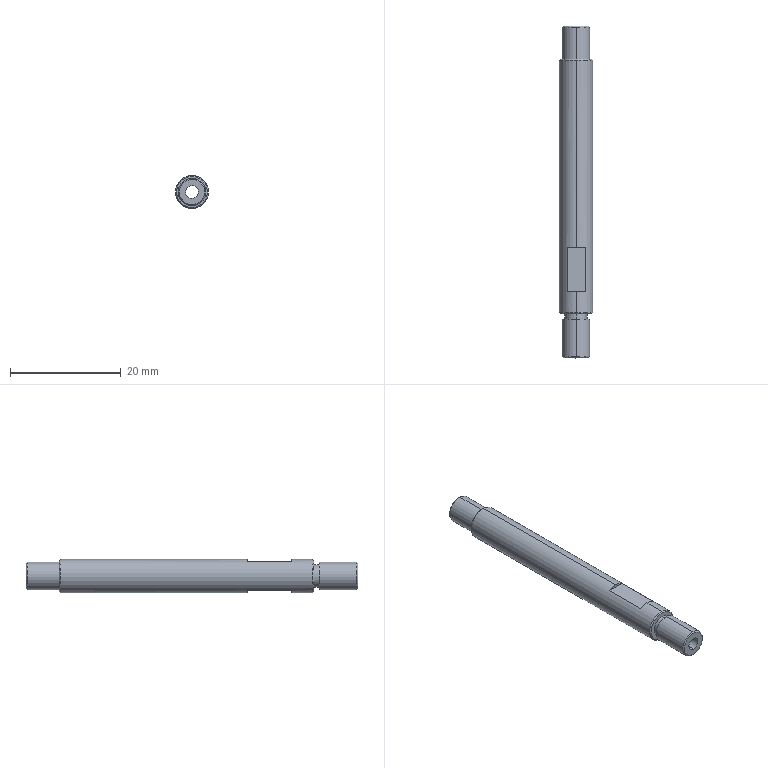Component | SolidWorks | F12529-M5106-1 | 1 solid | 29 faces | box 6 x 60 x 6 mm | volume 1300 mm3 | plane 11 | cylinder 10 | cone 8 | commonest cylinder face diameters 5 x4 2.3 x2 4 x2 6 x2 | material AISI 304
build123d program:
from build123d import *

# Parameters (mm, degrees)
SKETCH2_R          = 3
EXTRUDE1_DEPTH     = 52
SKETCH6_OUTSIDE_W  = 18.538
SKETCH6_OUTSIDE_H  = 18.538
SKETCH6_OUTSIDE_R  = 2.5
CUT_EXTRUDE2_DEPTH = 6
SKETCH7_R          = 2.5
EXTRUDE2_DEPTH     = 8
CHAMFER1_SIZE      = 0.2
SKETCH8_OUTSIDE_W  = 20.12
SKETCH8_OUTSIDE_H  = 20.12
SKETCH8_OUTSIDE_R  = 2
CUT_EXTRUDE3_DEPTH = 1
SKETCH9_R          = 1.15
CUT_EXTRUDE4_DEPTH = 61.15
CUT_EXTRUDE5_START = 2.5
SKETCH10_W         = 8
SKETCH10_H         = 8
CUT_EXTRUDE5_DEPTH = 10


with BuildPart() as part:
    # Sketch2 → Extrude1 (new body)
    with BuildSketch(Plane(origin=(0, 0, 0), x_dir=(1, 0, 0), z_dir=(0, 1, 0))):
        with Locations(Location((0, 0, 0), (0, 0, 90))):
            Circle(SKETCH2_R)
    extrude(amount=EXTRUDE1_DEPTH)

    # Sketch6 outside → Cut-Extrude2 (cut)
    with BuildSketch(Plane(origin=(0, 52, 0), x_dir=(1, 0, 0), z_dir=(0, 1, 0))):
        Rectangle(SKETCH6_OUTSIDE_W, SKETCH6_OUTSIDE_H)
        with Locations(Location((0, 0, 0), (0, 0, 270))):
            Circle(SKETCH6_OUTSIDE_R, mode=Mode.SUBTRACT)
    extrude(amount=-CUT_EXTRUDE2_DEPTH, mode=Mode.SUBTRACT)

    # Sketch7 → Extrude2 (add)
    with BuildSketch(Plane.XZ):
        with Locations(Location((0, 0, 0), (0, 0, 90))):
            Circle(SKETCH7_R)
    extrude(amount=EXTRUDE2_DEPTH)

    # Chamfer1
    chamfer1_edges = [part.edges().sort_by_distance(p)[0] for p in [
        (0, 52, -2.5),
        (0, 0, 3),
        (0, -8, -2.5),
        (0, 46, 3),
    ]]
    chamfer(chamfer1_edges, length=CHAMFER1_SIZE)

    # Sketch8 outside → Cut-Extrude3 (cut)
    with BuildSketch(Plane.XZ):
        Rectangle(SKETCH8_OUTSIDE_W, SKETCH8_OUTSIDE_H)
        with Locations(Location((0, 0, 0), (0, 0, 270))):
            Circle(SKETCH8_OUTSIDE_R, mode=Mode.SUBTRACT)
    extrude(amount=CUT_EXTRUDE3_DEPTH, mode=Mode.SUBTRACT)

    # Sketch9 → Cut-Extrude4 (cut, through all)
    with BuildSketch(Plane(origin=(0, 52, 0), x_dir=(1, 0, 0), z_dir=(0, 1, 0))):
        with Locations(Location((0, 0, 0), (0, 0, 270))):
            Circle(SKETCH9_R)
    extrude(amount=-CUT_EXTRUDE4_DEPTH, mode=Mode.SUBTRACT)

    # Sketch10 → Cut-Extrude5 (cut)
    with BuildSketch(Plane.XY.offset(CUT_EXTRUDE5_START)):
        with Locations((0, 8)):
            Rectangle(SKETCH10_W, SKETCH10_H)
    cut_extrude5 = extrude(amount=CUT_EXTRUDE5_DEPTH, mode=Mode.SUBTRACT)

    # Mirror1: Cut-Extrude5 across plane
    add(cut_extrude5.mirror(Plane.XY), mode=Mode.SUBTRACT)


solid = part.part

# Placed as in the assembly
solid = solid.moved(Location((-17.5, 227.5, 10), (180, -2.312, 180)))
STEP:
#1=CARTESIAN_POINT('',(-0.6908,8.642,0.3485));
#2=VERTEX_POINT('',#1);
#3=CARTESIAN_POINT('',(-0.6871,8.642,0.4389));
#4=VERTEX_POINT('',#3);
#5=CARTESIAN_POINT('',(-0.689,8.642,0.3937));
#6=DIRECTION('',(0.,1.,-0.));
#7=DIRECTION('',(0.04034,0.,0.9992));
#8=AXIS2_PLACEMENT_3D('',#5,#6,#7);
#9=CIRCLE('',#8,0.04528);
#10=EDGE_CURVE('',#2,#4,#9,.T.);
#11=ORIENTED_EDGE('',*,*,#10,.F.);
#12=CARTESIAN_POINT('',(-0.6908,11.004,0.3485));
#13=VERTEX_POINT('',#12);
#14=CARTESIAN_POINT('',(-0.6908,8.642,0.3485));
#15=DIRECTION('',(0.,1.,-0.));
#16=VECTOR('',#15,39.37);
#17=LINE('',#14,#16);
#18=EDGE_CURVE('',#2,#13,#17,.T.);
#19=ORIENTED_EDGE('',*,*,#18,.T.);
#20=CARTESIAN_POINT('',(-0.6871,11.004,0.4389));
#21=VERTEX_POINT('',#20);
#22=CARTESIAN_POINT('',(-0.689,11.004,0.3937));
#23=DIRECTION('',(0.,1.,-0.));
#24=DIRECTION('',(0.04034,0.,0.9992));
#25=AXIS2_PLACEMENT_3D('',#22,#23,#24);
#26=CIRCLE('',#25,0.04528);
#27=EDGE_CURVE('',#13,#21,#26,.T.);
#28=ORIENTED_EDGE('',*,*,#27,.T.);
#29=CARTESIAN_POINT('',(-0.6871,8.642,0.4389));
#30=DIRECTION('',(0.,1.,-0.));
#31=VECTOR('',#30,39.37);
#32=LINE('',#29,#31);
#33=EDGE_CURVE('',#4,#21,#32,.T.);
#34=ORIENTED_EDGE('',*,*,#33,.F.);
#35=EDGE_LOOP('',(#11,#19,#28,#34));
#36=FACE_OUTER_BOUND('',#35,.T.);
#37=CARTESIAN_POINT('',(-0.689,8.642,0.3937));
#38=DIRECTION('',(0.,1.,-0.));
#39=DIRECTION('',(0.04034,0.,0.9992));
#40=AXIS2_PLACEMENT_3D('',#37,#38,#39);
#41=CYLINDRICAL_SURFACE('',#40,0.04528);
#42=ADVANCED_FACE('',(#36),#41,.F.);
#43=CARTESIAN_POINT('',(-0.685,8.65,0.492));
#44=VERTEX_POINT('',#43);
#45=CARTESIAN_POINT('',(-0.6929,8.65,0.2954));
#46=VERTEX_POINT('',#45);
#47=CARTESIAN_POINT('',(-0.689,8.65,0.3937));
#48=DIRECTION('',(0.,1.,-0.));
#49=DIRECTION('',(-0.04034,0.,-0.9992));
#50=AXIS2_PLACEMENT_3D('',#47,#48,#49);
#51=CIRCLE('',#50,0.09843);
#52=EDGE_CURVE('',#44,#46,#51,.T.);
#53=ORIENTED_EDGE('',*,*,#52,.T.);
#54=CARTESIAN_POINT('',(-0.6929,8.917,0.2954));
#55=VERTEX_POINT('',#54);
#56=CARTESIAN_POINT('',(-0.6929,8.642,0.2954));
#57=DIRECTION('',(0.,1.,-0.));
#58=VECTOR('',#57,39.37);
#59=LINE('',#56,#58);
#60=EDGE_CURVE('',#46,#55,#59,.T.);
#61=ORIENTED_EDGE('',*,*,#60,.T.);
#62=CARTESIAN_POINT('',(-0.685,8.917,0.492));
#63=VERTEX_POINT('',#62);
#64=CARTESIAN_POINT('',(-0.689,8.917,0.3937));
#65=DIRECTION('',(-0.,-1.,0.));
#66=DIRECTION('',(-0.04034,0.,-0.9992));
#67=AXIS2_PLACEMENT_3D('',#64,#65,#66);
#68=CIRCLE('',#67,0.09843);
#69=EDGE_CURVE('',#55,#63,#68,.T.);
#70=ORIENTED_EDGE('',*,*,#69,.T.);
#71=CARTESIAN_POINT('',(-0.685,8.642,0.492));
#72=DIRECTION('',(0.,1.,-0.));
#73=VECTOR('',#72,39.37);
#74=LINE('',#71,#73);
#75=EDGE_CURVE('',#44,#63,#74,.T.);
#76=ORIENTED_EDGE('',*,*,#75,.F.);
#77=EDGE_LOOP('',(#53,#61,#70,#76));
#78=FACE_OUTER_BOUND('',#77,.T.);
#79=CARTESIAN_POINT('',(-0.689,8.642,0.3937));
#80=DIRECTION('',(0.,1.,-0.));
#81=DIRECTION('',(0.04034,0.,0.9992));
#82=AXIS2_PLACEMENT_3D('',#79,#80,#81);
#83=CYLINDRICAL_SURFACE('',#82,0.09843);
#84=ADVANCED_FACE('',(#78),#83,.T.);
#85=CARTESIAN_POINT('',(-0.6926,8.642,0.3032));
#86=VERTEX_POINT('',#85);
#87=CARTESIAN_POINT('',(-0.6853,8.642,0.4842));
#88=VERTEX_POINT('',#87);
#89=CARTESIAN_POINT('',(-0.689,8.642,0.3937));
#90=DIRECTION('',(-0.,-1.,0.));
#91=DIRECTION('',(-0.04034,0.,-0.9992));
#92=AXIS2_PLACEMENT_3D('',#89,#90,#91);
#93=CIRCLE('',#92,0.09055);
#94=EDGE_CURVE('',#86,#88,#93,.T.);
#95=ORIENTED_EDGE('',*,*,#94,.F.);
#96=CARTESIAN_POINT('',(-0.6926,8.642,0.3032));
#97=DIRECTION('',(-0.02853,0.7071,-0.7065));
#98=VECTOR('',#97,39.37);
#99=LINE('',#96,#98);
#100=EDGE_CURVE('',#86,#46,#99,.T.);
#101=ORIENTED_EDGE('',*,*,#100,.T.);
#102=ORIENTED_EDGE('',*,*,#52,.F.);
#103=CARTESIAN_POINT('',(-0.6853,8.642,0.4842));
#104=DIRECTION('',(0.02853,0.7071,0.7065));
#105=VECTOR('',#104,39.37);
#106=LINE('',#103,#105);
#107=EDGE_CURVE('',#88,#44,#106,.T.);
#108=ORIENTED_EDGE('',*,*,#107,.F.);
#109=EDGE_LOOP('',(#95,#101,#102,#108));
#110=FACE_OUTER_BOUND('',#109,.T.);
#111=CARTESIAN_POINT('',(-0.689,8.642,0.3937));
#112=DIRECTION('',(0.,1.,-0.));
#113=DIRECTION('',(0.04034,0.,0.9992));
#114=AXIS2_PLACEMENT_3D('',#111,#112,#113);
#115=CONICAL_SURFACE('',#114,0.09055,0.7854);
#116=ADVANCED_FACE('',(#110),#115,.T.);
#117=CARTESIAN_POINT('',(-0.6922,8.917,0.315));
#118=VERTEX_POINT('',#117);
#119=CARTESIAN_POINT('',(-0.6858,8.917,0.4724));
#120=VERTEX_POINT('',#119);
#121=CARTESIAN_POINT('',(-0.689,8.917,0.3937));
#122=DIRECTION('',(-0.,-1.,0.));
#123=DIRECTION('',(-0.04034,0.,-0.9992));
#124=AXIS2_PLACEMENT_3D('',#121,#122,#123);
#125=CIRCLE('',#124,0.07874);
#126=EDGE_CURVE('',#118,#120,#125,.T.);
#127=ORIENTED_EDGE('',*,*,#126,.F.);
#128=CARTESIAN_POINT('',(-0.6922,8.957,0.315));
#129=VERTEX_POINT('',#128);
#130=CARTESIAN_POINT('',(-0.6922,8.917,0.315));
#131=DIRECTION('',(0.,1.,-0.));
#132=VECTOR('',#131,39.37);
#133=LINE('',#130,#132);
#134=EDGE_CURVE('',#118,#129,#133,.T.);
#135=ORIENTED_EDGE('',*,*,#134,.T.);
#136=CARTESIAN_POINT('',(-0.6858,8.957,0.4724));
#137=VERTEX_POINT('',#136);
#138=CARTESIAN_POINT('',(-0.689,8.957,0.3937));
#139=DIRECTION('',(-0.,-1.,0.));
#140=DIRECTION('',(-0.04034,0.,-0.9992));
#141=AXIS2_PLACEMENT_3D('',#138,#139,#140);
#142=CIRCLE('',#141,0.07874);
#143=EDGE_CURVE('',#129,#137,#142,.T.);
#144=ORIENTED_EDGE('',*,*,#143,.T.);
#145=CARTESIAN_POINT('',(-0.6858,8.917,0.4724));
#146=DIRECTION('',(0.,1.,-0.));
#147=VECTOR('',#146,39.37);
#148=LINE('',#145,#147);
#149=EDGE_CURVE('',#120,#137,#148,.T.);
#150=ORIENTED_EDGE('',*,*,#149,.F.);
#151=EDGE_LOOP('',(#127,#135,#144,#150));
#152=FACE_OUTER_BOUND('',#151,.T.);
#153=CARTESIAN_POINT('',(-0.689,8.917,0.3937));
#154=DIRECTION('',(0.,1.,-0.));
#155=DIRECTION('',(0.04034,0.,0.9992));
#156=AXIS2_PLACEMENT_3D('',#153,#154,#155);
#157=CYLINDRICAL_SURFACE('',#156,0.07874);
#158=ADVANCED_FACE('',(#152),#157,.T.);
#159=CARTESIAN_POINT('',(-0.6853,11.004,0.4842));
#160=VERTEX_POINT('',#159);
#161=CARTESIAN_POINT('',(-0.6926,11.004,0.3032));
#162=VERTEX_POINT('',#161);
#163=CARTESIAN_POINT('',(-0.689,11.004,0.3937));
#164=DIRECTION('',(0.,1.,-0.));
#165=DIRECTION('',(0.04034,0.,0.9992));
#166=AXIS2_PLACEMENT_3D('',#163,#164,#165);
#167=CIRCLE('',#166,0.09055);
#168=EDGE_CURVE('',#160,#162,#167,.T.);
#169=ORIENTED_EDGE('',*,*,#168,.F.);
#170=CARTESIAN_POINT('',(-0.685,10.996,0.492));
#171=VERTEX_POINT('',#170);
#172=CARTESIAN_POINT('',(-0.6853,11.004,0.4842));
#173=DIRECTION('',(0.02853,-0.7071,0.7065));
#174=VECTOR('',#173,39.37);
#175=LINE('',#172,#174);
#176=EDGE_CURVE('',#160,#171,#175,.T.);
#177=ORIENTED_EDGE('',*,*,#176,.T.);
#178=CARTESIAN_POINT('',(-0.6929,10.996,0.2954));
#179=VERTEX_POINT('',#178);
#180=CARTESIAN_POINT('',(-0.689,10.996,0.3937));
#181=DIRECTION('',(-0.,-1.,0.));
#182=DIRECTION('',(0.04034,0.,0.9992));
#183=AXIS2_PLACEMENT_3D('',#180,#181,#182);
#184=CIRCLE('',#183,0.09843);
#185=EDGE_CURVE('',#179,#171,#184,.T.);
#186=ORIENTED_EDGE('',*,*,#185,.F.);
#187=CARTESIAN_POINT('',(-0.6926,11.004,0.3032));
#188=DIRECTION('',(-0.02853,-0.7071,-0.7065));
#189=VECTOR('',#188,39.37);
#190=LINE('',#187,#189);
#191=EDGE_CURVE('',#162,#179,#190,.T.);
#192=ORIENTED_EDGE('',*,*,#191,.F.);
#193=EDGE_LOOP('',(#169,#177,#186,#192));
#194=FACE_OUTER_BOUND('',#193,.T.);
#195=CARTESIAN_POINT('',(-0.689,11.004,0.3937));
#196=DIRECTION('',(-0.,-1.,0.));
#197=DIRECTION('',(-0.04034,0.,-0.9992));
#198=AXIS2_PLACEMENT_3D('',#195,#196,#197);
#199=CONICAL_SURFACE('',#198,0.09055,0.7854);
#200=ADVANCED_FACE('',(#194),#199,.T.);
#201=CARTESIAN_POINT('',(-0.6845,10.768,0.5038));
#202=VERTEX_POINT('',#201);
#203=CARTESIAN_POINT('',(-0.6934,10.768,0.2836));
#204=VERTEX_POINT('',#203);
#205=CARTESIAN_POINT('',(-0.689,10.768,0.3937));
#206=DIRECTION('',(0.,1.,-0.));
#207=DIRECTION('',(0.04034,0.,0.9992));
#208=AXIS2_PLACEMENT_3D('',#205,#206,#207);
#209=CIRCLE('',#208,0.1102);
#210=EDGE_CURVE('',#202,#204,#209,.T.);
#211=ORIENTED_EDGE('',*,*,#210,.F.);
#212=CARTESIAN_POINT('',(-0.6842,10.76,0.5117));
#213=VERTEX_POINT('',#212);
#214=CARTESIAN_POINT('',(-0.6845,10.768,0.5038));
#215=DIRECTION('',(0.02853,-0.7071,0.7065));
#216=VECTOR('',#215,39.37);
#217=LINE('',#214,#216);
#218=EDGE_CURVE('',#202,#213,#217,.T.);
#219=ORIENTED_EDGE('',*,*,#218,.T.);
#220=CARTESIAN_POINT('',(-0.6937,10.76,0.2757));
#221=VERTEX_POINT('',#220);
#222=CARTESIAN_POINT('',(-0.689,10.76,0.3937));
#223=DIRECTION('',(-0.,-1.,0.));
#224=DIRECTION('',(0.04034,0.,0.9992));
#225=AXIS2_PLACEMENT_3D('',#222,#223,#224);
#226=CIRCLE('',#225,0.1181);
#227=EDGE_CURVE('',#221,#213,#226,.T.);
#228=ORIENTED_EDGE('',*,*,#227,.F.);
#229=CARTESIAN_POINT('',(-0.6934,10.768,0.2836));
#230=DIRECTION('',(-0.02853,-0.7071,-0.7065));
#231=VECTOR('',#230,39.37);
#232=LINE('',#229,#231);
#233=EDGE_CURVE('',#204,#221,#232,.T.);
#234=ORIENTED_EDGE('',*,*,#233,.F.);
#235=EDGE_LOOP('',(#211,#219,#228,#234));
#236=FACE_OUTER_BOUND('',#235,.T.);
#237=CARTESIAN_POINT('',(-0.689,10.768,0.3937));
#238=DIRECTION('',(-0.,-1.,0.));
#239=DIRECTION('',(-0.04034,0.,-0.9992));
#240=AXIS2_PLACEMENT_3D('',#237,#238,#239);
#241=CONICAL_SURFACE('',#240,0.1102,0.7854);
#242=ADVANCED_FACE('',(#236),#241,.T.);
#243=CARTESIAN_POINT('',(-0.6934,8.957,0.2836));
#244=VERTEX_POINT('',#243);
#245=CARTESIAN_POINT('',(-0.6845,8.957,0.5038));
#246=VERTEX_POINT('',#245);
#247=CARTESIAN_POINT('',(-0.689,8.957,0.3937));
#248=DIRECTION('',(-0.,-1.,0.));
#249=DIRECTION('',(0.04034,0.,0.9992));
#250=AXIS2_PLACEMENT_3D('',#247,#248,#249);
#251=CIRCLE('',#250,0.1102);
#252=EDGE_CURVE('',#244,#246,#251,.T.);
#253=ORIENTED_EDGE('',*,*,#252,.F.);
#254=CARTESIAN_POINT('',(-0.6937,8.965,0.2757));
#255=VERTEX_POINT('',#254);
#256=CARTESIAN_POINT('',(-0.6937,8.965,0.2757));
#257=DIRECTION('',(-0.02853,0.7071,-0.7065));
#258=VECTOR('',#257,39.37);
#259=LINE('',#256,#258);
#260=EDGE_CURVE('',#244,#255,#259,.T.);
#261=ORIENTED_EDGE('',*,*,#260,.T.);
#262=CARTESIAN_POINT('',(-0.6842,8.965,0.5117));
#263=VERTEX_POINT('',#262);
#264=CARTESIAN_POINT('',(-0.689,8.965,0.3937));
#265=DIRECTION('',(0.,1.,-0.));
#266=DIRECTION('',(0.04034,0.,0.9992));
#267=AXIS2_PLACEMENT_3D('',#264,#265,#266);
#268=CIRCLE('',#267,0.1181);
#269=EDGE_CURVE('',#263,#255,#268,.T.);
#270=ORIENTED_EDGE('',*,*,#269,.F.);
#271=CARTESIAN_POINT('',(-0.6842,8.965,0.5117));
#272=DIRECTION('',(0.02853,0.7071,0.7065));
#273=VECTOR('',#272,39.37);
#274=LINE('',#271,#273);
#275=EDGE_CURVE('',#246,#263,#274,.T.);
#276=ORIENTED_EDGE('',*,*,#275,.F.);
#277=EDGE_LOOP('',(#253,#261,#270,#276));
#278=FACE_OUTER_BOUND('',#277,.T.);
#279=CARTESIAN_POINT('',(-0.689,8.965,0.3937));
#280=DIRECTION('',(0.,1.,-0.));
#281=DIRECTION('',(0.04034,0.,0.9992));
#282=AXIS2_PLACEMENT_3D('',#279,#280,#281);
#283=CONICAL_SURFACE('',#282,0.1181,0.7854);
#284=ADVANCED_FACE('',(#278),#283,.T.);
#285=CARTESIAN_POINT('',(-0.685,10.768,0.492));
#286=VERTEX_POINT('',#285);
#287=CARTESIAN_POINT('',(-0.6929,10.768,0.2954));
#288=VERTEX_POINT('',#287);
#289=CARTESIAN_POINT('',(-0.689,10.768,0.3937));
#290=DIRECTION('',(0.,1.,-0.));
#291=DIRECTION('',(0.04034,0.,0.9992));
#292=AXIS2_PLACEMENT_3D('',#289,#290,#291);
#293=CIRCLE('',#292,0.09843);
#294=EDGE_CURVE('',#286,#288,#293,.T.);
#295=ORIENTED_EDGE('',*,*,#294,.T.);
#296=CARTESIAN_POINT('',(-0.6929,10.768,0.2954));
#297=DIRECTION('',(0.,1.,-0.));
#298=VECTOR('',#297,39.37);
#299=LINE('',#296,#298);
#300=EDGE_CURVE('',#288,#179,#299,.T.);
#301=ORIENTED_EDGE('',*,*,#300,.T.);
#302=ORIENTED_EDGE('',*,*,#185,.T.);
#303=CARTESIAN_POINT('',(-0.685,10.768,0.492));
#304=DIRECTION('',(0.,1.,-0.));
#305=VECTOR('',#304,39.37);
#306=LINE('',#303,#305);
#307=EDGE_CURVE('',#286,#171,#306,.T.);
#308=ORIENTED_EDGE('',*,*,#307,.F.);
#309=EDGE_LOOP('',(#295,#301,#302,#308));
#310=FACE_OUTER_BOUND('',#309,.T.);
#311=CARTESIAN_POINT('',(-0.689,10.768,0.3937));
#312=DIRECTION('',(0.,1.,-0.));
#313=DIRECTION('',(0.04034,0.,0.9992));
#314=AXIS2_PLACEMENT_3D('',#311,#312,#313);
#315=CYLINDRICAL_SURFACE('',#314,0.09843);
#316=ADVANCED_FACE('',(#310),#315,.T.);
#317=ORIENTED_EDGE('',*,*,#227,.T.);
#318=CARTESIAN_POINT('',(-0.6842,9.429,0.5117));
#319=VERTEX_POINT('',#318);
#320=CARTESIAN_POINT('',(-0.6842,11.004,0.5117));
#321=DIRECTION('',(-0.,-1.,0.));
#322=VECTOR('',#321,39.37);
#323=LINE('',#320,#322);
#324=EDGE_CURVE('',#213,#319,#323,.T.);
#325=ORIENTED_EDGE('',*,*,#324,.T.);
#326=CARTESIAN_POINT('',(-0.6198,9.429,0.4894));
#327=VERTEX_POINT('',#326);
#328=CARTESIAN_POINT('',(-0.689,9.429,0.3937));
#329=DIRECTION('',(-0.,-1.,0.));
#330=DIRECTION('',(-0.04034,0.,-0.9992));
#331=AXIS2_PLACEMENT_3D('',#328,#329,#330);
#332=CIRCLE('',#331,0.1181);
#333=EDGE_CURVE('',#327,#319,#332,.T.);
#334=ORIENTED_EDGE('',*,*,#333,.F.);
#335=CARTESIAN_POINT('',(-0.6198,9.114,0.4894));
#336=VERTEX_POINT('',#335);
#337=CARTESIAN_POINT('',(-0.6198,11.004,0.4894));
#338=DIRECTION('',(0.,1.,-0.));
#339=VECTOR('',#338,39.37);
#340=LINE('',#337,#339);
#341=EDGE_CURVE('',#336,#327,#340,.T.);
#342=ORIENTED_EDGE('',*,*,#341,.F.);
#343=CARTESIAN_POINT('',(-0.6842,9.114,0.5117));
#344=VERTEX_POINT('',#343);
#345=CARTESIAN_POINT('',(-0.689,9.114,0.3937));
#346=DIRECTION('',(0.,1.,-0.));
#347=DIRECTION('',(0.04034,0.,0.9992));
#348=AXIS2_PLACEMENT_3D('',#345,#346,#347);
#349=CIRCLE('',#348,0.1181);
#350=EDGE_CURVE('',#344,#336,#349,.T.);
#351=ORIENTED_EDGE('',*,*,#350,.F.);
#352=CARTESIAN_POINT('',(-0.6842,11.004,0.5117));
#353=DIRECTION('',(-0.,-1.,0.));
#354=VECTOR('',#353,39.37);
#355=LINE('',#352,#354);
#356=EDGE_CURVE('',#344,#263,#355,.T.);
#357=ORIENTED_EDGE('',*,*,#356,.T.);
#358=ORIENTED_EDGE('',*,*,#269,.T.);
#359=CARTESIAN_POINT('',(-0.6937,9.114,0.2757));
#360=VERTEX_POINT('',#359);
#361=CARTESIAN_POINT('',(-0.6937,11.004,0.2757));
#362=DIRECTION('',(-0.,-1.,0.));
#363=VECTOR('',#362,39.37);
#364=LINE('',#361,#363);
#365=EDGE_CURVE('',#360,#255,#364,.T.);
#366=ORIENTED_EDGE('',*,*,#365,.F.);
#367=CARTESIAN_POINT('',(-0.6277,9.114,0.2927));
#368=VERTEX_POINT('',#367);
#369=CARTESIAN_POINT('',(-0.689,9.114,0.3937));
#370=DIRECTION('',(-0.,-1.,0.));
#371=DIRECTION('',(-0.04034,0.,-0.9992));
#372=AXIS2_PLACEMENT_3D('',#369,#370,#371);
#373=CIRCLE('',#372,0.1181);
#374=EDGE_CURVE('',#360,#368,#373,.T.);
#375=ORIENTED_EDGE('',*,*,#374,.T.);
#376=CARTESIAN_POINT('',(-0.6277,9.429,0.2927));
#377=VERTEX_POINT('',#376);
#378=CARTESIAN_POINT('',(-0.6277,11.004,0.2927));
#379=DIRECTION('',(-0.,-1.,0.));
#380=VECTOR('',#379,39.37);
#381=LINE('',#378,#380);
#382=EDGE_CURVE('',#377,#368,#381,.T.);
#383=ORIENTED_EDGE('',*,*,#382,.F.);
#384=CARTESIAN_POINT('',(-0.6937,9.429,0.2757));
#385=VERTEX_POINT('',#384);
#386=CARTESIAN_POINT('',(-0.689,9.429,0.3937));
#387=DIRECTION('',(0.,1.,-0.));
#388=DIRECTION('',(0.04034,0.,0.9992));
#389=AXIS2_PLACEMENT_3D('',#386,#387,#388);
#390=CIRCLE('',#389,0.1181);
#391=EDGE_CURVE('',#377,#385,#390,.T.);
#392=ORIENTED_EDGE('',*,*,#391,.T.);
#393=CARTESIAN_POINT('',(-0.6937,11.004,0.2757));
#394=DIRECTION('',(-0.,-1.,0.));
#395=VECTOR('',#394,39.37);
#396=LINE('',#393,#395);
#397=EDGE_CURVE('',#221,#385,#396,.T.);
#398=ORIENTED_EDGE('',*,*,#397,.F.);
#399=EDGE_LOOP('',(#317,#325,#334,#342,#351,#357,#358,#366,#375,#383,#392,#398));
#400=FACE_OUTER_BOUND('',#399,.T.);
#401=CARTESIAN_POINT('',(-0.689,11.004,0.3937));
#402=DIRECTION('',(-0.,-1.,0.));
#403=DIRECTION('',(-0.04034,0.,-0.9992));
#404=AXIS2_PLACEMENT_3D('',#401,#402,#403);
#405=CYLINDRICAL_SURFACE('',#404,0.1181);
#406=ADVANCED_FACE('',(#400),#405,.T.);
#407=ORIENTED_EDGE('',*,*,#324,.F.);
#408=CARTESIAN_POINT('',(-0.689,10.76,0.3937));
#409=DIRECTION('',(-0.,-1.,0.));
#410=DIRECTION('',(0.04034,0.,0.9992));
#411=AXIS2_PLACEMENT_3D('',#408,#409,#410);
#412=CIRCLE('',#411,0.1181);
#413=EDGE_CURVE('',#213,#221,#412,.T.);
#414=ORIENTED_EDGE('',*,*,#413,.T.);
#415=ORIENTED_EDGE('',*,*,#397,.T.);
#416=CARTESIAN_POINT('',(-0.7582,9.429,0.298));
#417=VERTEX_POINT('',#416);
#418=CARTESIAN_POINT('',(-0.689,9.429,0.3937));
#419=DIRECTION('',(0.,1.,-0.));
#420=DIRECTION('',(0.04034,0.,0.9992));
#421=AXIS2_PLACEMENT_3D('',#418,#419,#420);
#422=CIRCLE('',#421,0.1181);
#423=EDGE_CURVE('',#385,#417,#422,.T.);
#424=ORIENTED_EDGE('',*,*,#423,.T.);
#425=CARTESIAN_POINT('',(-0.7582,9.114,0.298));
#426=VERTEX_POINT('',#425);
#427=CARTESIAN_POINT('',(-0.7582,11.004,0.298));
#428=DIRECTION('',(0.,1.,-0.));
#429=VECTOR('',#428,39.37);
#430=LINE('',#427,#429);
#431=EDGE_CURVE('',#426,#417,#430,.T.);
#432=ORIENTED_EDGE('',*,*,#431,.F.);
#433=CARTESIAN_POINT('',(-0.689,9.114,0.3937));
#434=DIRECTION('',(-0.,-1.,0.));
#435=DIRECTION('',(-0.04034,0.,-0.9992));
#436=AXIS2_PLACEMENT_3D('',#433,#434,#435);
#437=CIRCLE('',#436,0.1181);
#438=EDGE_CURVE('',#426,#360,#437,.T.);
#439=ORIENTED_EDGE('',*,*,#438,.T.);
#440=ORIENTED_EDGE('',*,*,#365,.T.);
#441=CARTESIAN_POINT('',(-0.689,8.965,0.3937));
#442=DIRECTION('',(0.,1.,-0.));
#443=DIRECTION('',(0.04034,0.,0.9992));
#444=AXIS2_PLACEMENT_3D('',#441,#442,#443);
#445=CIRCLE('',#444,0.1181);
#446=EDGE_CURVE('',#255,#263,#445,.T.);
#447=ORIENTED_EDGE('',*,*,#446,.T.);
#448=ORIENTED_EDGE('',*,*,#356,.F.);
#449=CARTESIAN_POINT('',(-0.7502,9.114,0.4947));
#450=VERTEX_POINT('',#449);
#451=CARTESIAN_POINT('',(-0.689,9.114,0.3937));
#452=DIRECTION('',(0.,1.,-0.));
#453=DIRECTION('',(0.04034,0.,0.9992));
#454=AXIS2_PLACEMENT_3D('',#451,#452,#453);
#455=CIRCLE('',#454,0.1181);
#456=EDGE_CURVE('',#450,#344,#455,.T.);
#457=ORIENTED_EDGE('',*,*,#456,.F.);
#458=CARTESIAN_POINT('',(-0.7502,9.429,0.4947));
#459=VERTEX_POINT('',#458);
#460=CARTESIAN_POINT('',(-0.7502,11.004,0.4947));
#461=DIRECTION('',(-0.,-1.,0.));
#462=VECTOR('',#461,39.37);
#463=LINE('',#460,#462);
#464=EDGE_CURVE('',#459,#450,#463,.T.);
#465=ORIENTED_EDGE('',*,*,#464,.F.);
#466=CARTESIAN_POINT('',(-0.689,9.429,0.3937));
#467=DIRECTION('',(-0.,-1.,0.));
#468=DIRECTION('',(-0.04034,0.,-0.9992));
#469=AXIS2_PLACEMENT_3D('',#466,#467,#468);
#470=CIRCLE('',#469,0.1181);
#471=EDGE_CURVE('',#319,#459,#470,.T.);
#472=ORIENTED_EDGE('',*,*,#471,.F.);
#473=EDGE_LOOP('',(#407,#414,#415,#424,#432,#439,#440,#447,#448,#457,#465,#472));
#474=FACE_OUTER_BOUND('',#473,.T.);
#475=CARTESIAN_POINT('',(-0.689,11.004,0.3937));
#476=DIRECTION('',(-0.,-1.,0.));
#477=DIRECTION('',(-0.04034,0.,-0.9992));
#478=AXIS2_PLACEMENT_3D('',#475,#476,#477);
#479=CYLINDRICAL_SURFACE('',#478,0.1181);
#480=ADVANCED_FACE('',(#474),#479,.T.);
#481=CARTESIAN_POINT('',(-0.689,8.957,0.3937));
#482=DIRECTION('',(-0.,-1.,0.));
#483=DIRECTION('',(0.04034,0.,0.9992));
#484=AXIS2_PLACEMENT_3D('',#481,#482,#483);
#485=CIRCLE('',#484,0.1102);
#486=EDGE_CURVE('',#246,#244,#485,.T.);
#487=ORIENTED_EDGE('',*,*,#486,.T.);
#488=ORIENTED_EDGE('',*,*,#252,.T.);
#489=EDGE_LOOP('',(#487,#488));
#490=FACE_OUTER_BOUND('',#489,.T.);
#491=CARTESIAN_POINT('',(-0.689,8.957,0.3937));
#492=DIRECTION('',(-0.,-1.,0.));
#493=DIRECTION('',(-0.04034,0.,-0.9992));
#494=AXIS2_PLACEMENT_3D('',#491,#492,#493);
#495=CIRCLE('',#494,0.07874);
#496=EDGE_CURVE('',#137,#129,#495,.T.);
#497=ORIENTED_EDGE('',*,*,#496,.F.);
#498=ORIENTED_EDGE('',*,*,#143,.F.);
#499=EDGE_LOOP('',(#497,#498));
#500=FACE_BOUND('',#499,.T.);
#501=CARTESIAN_POINT('',(-0.689,8.957,0.3937));
#502=DIRECTION('',(0.,1.,-0.));
#503=DIRECTION('',(0.04034,0.,0.9992));
#504=AXIS2_PLACEMENT_3D('',#501,#502,#503);
#505=PLANE('',#504);
#506=ADVANCED_FACE('',(#490,#500),#505,.F.);
#507=CARTESIAN_POINT('',(-0.689,10.768,0.3937));
#508=DIRECTION('',(0.,1.,-0.));
#509=DIRECTION('',(0.04034,0.,0.9992));
#510=AXIS2_PLACEMENT_3D('',#507,#508,#509);
#511=CIRCLE('',#510,0.1102);
#512=EDGE_CURVE('',#204,#202,#511,.T.);
#513=ORIENTED_EDGE('',*,*,#512,.T.);
#514=ORIENTED_EDGE('',*,*,#210,.T.);
#515=EDGE_LOOP('',(#513,#514));
#516=FACE_OUTER_BOUND('',#515,.T.);
#517=ORIENTED_EDGE('',*,*,#294,.F.);
#518=CARTESIAN_POINT('',(-0.689,10.768,0.3937));
#519=DIRECTION('',(0.,1.,-0.));
#520=DIRECTION('',(0.04034,0.,0.9992));
#521=AXIS2_PLACEMENT_3D('',#518,#519,#520);
#522=CIRCLE('',#521,0.09843);
#523=EDGE_CURVE('',#288,#286,#522,.T.);
#524=ORIENTED_EDGE('',*,*,#523,.F.);
#525=EDGE_LOOP('',(#517,#524));
#526=FACE_BOUND('',#525,.T.);
#527=CARTESIAN_POINT('',(-0.689,10.768,0.3937));
#528=DIRECTION('',(0.,1.,-0.));
#529=DIRECTION('',(0.04034,0.,0.9992));
#530=AXIS2_PLACEMENT_3D('',#527,#528,#529);
#531=PLANE('',#530);
#532=ADVANCED_FACE('',(#516,#526),#531,.T.);
#533=ORIENTED_EDGE('',*,*,#300,.F.);
#534=ORIENTED_EDGE('',*,*,#523,.T.);
#535=ORIENTED_EDGE('',*,*,#307,.T.);
#536=CARTESIAN_POINT('',(-0.689,10.996,0.3937));
#537=DIRECTION('',(-0.,-1.,0.));
#538=DIRECTION('',(0.04034,0.,0.9992));
#539=AXIS2_PLACEMENT_3D('',#536,#537,#538);
#540=CIRCLE('',#539,0.09843);
#541=EDGE_CURVE('',#171,#179,#540,.T.);
#542=ORIENTED_EDGE('',*,*,#541,.T.);
#543=EDGE_LOOP('',(#533,#534,#535,#542));
#544=FACE_OUTER_BOUND('',#543,.T.);
#545=CARTESIAN_POINT('',(-0.689,10.768,0.3937));
#546=DIRECTION('',(0.,1.,-0.));
#547=DIRECTION('',(0.04034,0.,0.9992));
#548=AXIS2_PLACEMENT_3D('',#545,#546,#547);
#549=CYLINDRICAL_SURFACE('',#548,0.09843);
#550=ADVANCED_FACE('',(#544),#549,.T.);
#551=CARTESIAN_POINT('',(-0.689,11.004,0.3937));
#552=DIRECTION('',(0.,1.,-0.));
#553=DIRECTION('',(0.04034,0.,0.9992));
#554=AXIS2_PLACEMENT_3D('',#551,#552,#553);
#555=CIRCLE('',#554,0.04528);
#556=EDGE_CURVE('',#21,#13,#555,.T.);
#557=ORIENTED_EDGE('',*,*,#556,.F.);
#558=ORIENTED_EDGE('',*,*,#27,.F.);
#559=EDGE_LOOP('',(#557,#558));
#560=FACE_BOUND('',#559,.T.);
#561=CARTESIAN_POINT('',(-0.689,11.004,0.3937));
#562=DIRECTION('',(0.,1.,-0.));
#563=DIRECTION('',(0.04034,0.,0.9992));
#564=AXIS2_PLACEMENT_3D('',#561,#562,#563);
#565=CIRCLE('',#564,0.09055);
#566=EDGE_CURVE('',#162,#160,#565,.T.);
#567=ORIENTED_EDGE('',*,*,#566,.T.);
#568=ORIENTED_EDGE('',*,*,#168,.T.);
#569=EDGE_LOOP('',(#567,#568));
#570=FACE_OUTER_BOUND('',#569,.T.);
#571=CARTESIAN_POINT('',(-0.689,11.004,0.3937));
#572=DIRECTION('',(0.,1.,-0.));
#573=DIRECTION('',(0.04034,0.,0.9992));
#574=AXIS2_PLACEMENT_3D('',#571,#572,#573);
#575=PLANE('',#574);
#576=ADVANCED_FACE('',(#560,#570),#575,.T.);
#577=ORIENTED_EDGE('',*,*,#260,.F.);
#578=ORIENTED_EDGE('',*,*,#486,.F.);
#579=ORIENTED_EDGE('',*,*,#275,.T.);
#580=ORIENTED_EDGE('',*,*,#446,.F.);
#581=EDGE_LOOP('',(#577,#578,#579,#580));
#582=FACE_OUTER_BOUND('',#581,.T.);
#583=CARTESIAN_POINT('',(-0.689,8.965,0.3937));
#584=DIRECTION('',(0.,1.,-0.));
#585=DIRECTION('',(0.04034,0.,0.9992));
#586=AXIS2_PLACEMENT_3D('',#583,#584,#585);
#587=CONICAL_SURFACE('',#586,0.1181,0.7854);
#588=ADVANCED_FACE('',(#582),#587,.T.);
#589=ORIENTED_EDGE('',*,*,#218,.F.);
#590=ORIENTED_EDGE('',*,*,#512,.F.);
#591=ORIENTED_EDGE('',*,*,#233,.T.);
#592=ORIENTED_EDGE('',*,*,#413,.F.);
#593=EDGE_LOOP('',(#589,#590,#591,#592));
#594=FACE_OUTER_BOUND('',#593,.T.);
#595=CARTESIAN_POINT('',(-0.689,10.768,0.3937));
#596=DIRECTION('',(-0.,-1.,0.));
#597=DIRECTION('',(-0.04034,0.,-0.9992));
#598=AXIS2_PLACEMENT_3D('',#595,#596,#597);
#599=CONICAL_SURFACE('',#598,0.1102,0.7854);
#600=ADVANCED_FACE('',(#594),#599,.T.);
#601=ORIENTED_EDGE('',*,*,#176,.F.);
#602=ORIENTED_EDGE('',*,*,#566,.F.);
#603=ORIENTED_EDGE('',*,*,#191,.T.);
#604=ORIENTED_EDGE('',*,*,#541,.F.);
#605=EDGE_LOOP('',(#601,#602,#603,#604));
#606=FACE_OUTER_BOUND('',#605,.T.);
#607=CARTESIAN_POINT('',(-0.689,11.004,0.3937));
#608=DIRECTION('',(-0.,-1.,0.));
#609=DIRECTION('',(-0.04034,0.,-0.9992));
#610=AXIS2_PLACEMENT_3D('',#607,#608,#609);
#611=CONICAL_SURFACE('',#610,0.09055,0.7854);
#612=ADVANCED_FACE('',(#606),#611,.T.);
#613=CARTESIAN_POINT('',(-0.689,8.917,0.3937));
#614=DIRECTION('',(-0.,-1.,0.));
#615=DIRECTION('',(-0.04034,0.,-0.9992));
#616=AXIS2_PLACEMENT_3D('',#613,#614,#615);
#617=CIRCLE('',#616,0.07874);
#618=EDGE_CURVE('',#120,#118,#617,.T.);
#619=ORIENTED_EDGE('',*,*,#618,.T.);
#620=ORIENTED_EDGE('',*,*,#126,.T.);
#621=EDGE_LOOP('',(#619,#620));
#622=FACE_BOUND('',#621,.T.);
#623=CARTESIAN_POINT('',(-0.689,8.917,0.3937));
#624=DIRECTION('',(-0.,-1.,0.));
#625=DIRECTION('',(-0.04034,0.,-0.9992));
#626=AXIS2_PLACEMENT_3D('',#623,#624,#625);
#627=CIRCLE('',#626,0.09843);
#628=EDGE_CURVE('',#63,#55,#627,.T.);
#629=ORIENTED_EDGE('',*,*,#628,.F.);
#630=ORIENTED_EDGE('',*,*,#69,.F.);
#631=EDGE_LOOP('',(#629,#630));
#632=FACE_OUTER_BOUND('',#631,.T.);
#633=CARTESIAN_POINT('',(-0.689,8.917,0.3937));
#634=DIRECTION('',(-0.,-1.,0.));
#635=DIRECTION('',(-0.04034,-0.,-0.9992));
#636=AXIS2_PLACEMENT_3D('',#633,#634,#635);
#637=PLANE('',#636);
#638=ADVANCED_FACE('',(#622,#632),#637,.F.);
#639=ORIENTED_EDGE('',*,*,#134,.F.);
#640=ORIENTED_EDGE('',*,*,#618,.F.);
#641=ORIENTED_EDGE('',*,*,#149,.T.);
#642=ORIENTED_EDGE('',*,*,#496,.T.);
#643=EDGE_LOOP('',(#639,#640,#641,#642));
#644=FACE_OUTER_BOUND('',#643,.T.);
#645=CARTESIAN_POINT('',(-0.689,8.917,0.3937));
#646=DIRECTION('',(0.,1.,-0.));
#647=DIRECTION('',(0.04034,0.,0.9992));
#648=AXIS2_PLACEMENT_3D('',#645,#646,#647);
#649=CYLINDRICAL_SURFACE('',#648,0.07874);
#650=ADVANCED_FACE('',(#644),#649,.T.);
#651=CARTESIAN_POINT('',(-0.689,8.642,0.3937));
#652=DIRECTION('',(0.,1.,-0.));
#653=DIRECTION('',(0.04034,0.,0.9992));
#654=AXIS2_PLACEMENT_3D('',#651,#652,#653);
#655=CIRCLE('',#654,0.04528);
#656=EDGE_CURVE('',#4,#2,#655,.T.);
#657=ORIENTED_EDGE('',*,*,#656,.T.);
#658=ORIENTED_EDGE('',*,*,#10,.T.);
#659=EDGE_LOOP('',(#657,#658));
#660=FACE_BOUND('',#659,.T.);
#661=CARTESIAN_POINT('',(-0.689,8.642,0.3937));
#662=DIRECTION('',(-0.,-1.,0.));
#663=DIRECTION('',(-0.04034,0.,-0.9992));
#664=AXIS2_PLACEMENT_3D('',#661,#662,#663);
#665=CIRCLE('',#664,0.09055);
#666=EDGE_CURVE('',#88,#86,#665,.T.);
#667=ORIENTED_EDGE('',*,*,#666,.T.);
#668=ORIENTED_EDGE('',*,*,#94,.T.);
#669=EDGE_LOOP('',(#667,#668));
#670=FACE_OUTER_BOUND('',#669,.T.);
#671=CARTESIAN_POINT('',(-0.689,8.642,0.3937));
#672=DIRECTION('',(-0.,-1.,0.));
#673=DIRECTION('',(-0.04034,-0.,-0.9992));
#674=AXIS2_PLACEMENT_3D('',#671,#672,#673);
#675=PLANE('',#674);
#676=ADVANCED_FACE('',(#660,#670),#675,.T.);
#677=ORIENTED_EDGE('',*,*,#100,.F.);
#678=ORIENTED_EDGE('',*,*,#666,.F.);
#679=ORIENTED_EDGE('',*,*,#107,.T.);
#680=CARTESIAN_POINT('',(-0.689,8.65,0.3937));
#681=DIRECTION('',(0.,1.,-0.));
#682=DIRECTION('',(-0.04034,0.,-0.9992));
#683=AXIS2_PLACEMENT_3D('',#680,#681,#682);
#684=CIRCLE('',#683,0.09843);
#685=EDGE_CURVE('',#46,#44,#684,.T.);
#686=ORIENTED_EDGE('',*,*,#685,.F.);
#687=EDGE_LOOP('',(#677,#678,#679,#686));
#688=FACE_OUTER_BOUND('',#687,.T.);
#689=CARTESIAN_POINT('',(-0.689,8.642,0.3937));
#690=DIRECTION('',(0.,1.,-0.));
#691=DIRECTION('',(0.04034,0.,0.9992));
#692=AXIS2_PLACEMENT_3D('',#689,#690,#691);
#693=CONICAL_SURFACE('',#692,0.09055,0.7854);
#694=ADVANCED_FACE('',(#688),#693,.T.);
#695=ORIENTED_EDGE('',*,*,#60,.F.);
#696=ORIENTED_EDGE('',*,*,#685,.T.);
#697=ORIENTED_EDGE('',*,*,#75,.T.);
#698=ORIENTED_EDGE('',*,*,#628,.T.);
#699=EDGE_LOOP('',(#695,#696,#697,#698));
#700=FACE_OUTER_BOUND('',#699,.T.);
#701=CARTESIAN_POINT('',(-0.689,8.642,0.3937));
#702=DIRECTION('',(0.,1.,-0.));
#703=DIRECTION('',(0.04034,0.,0.9992));
#704=AXIS2_PLACEMENT_3D('',#701,#702,#703);
#705=CYLINDRICAL_SURFACE('',#704,0.09843);
#706=ADVANCED_FACE('',(#700),#705,.T.);
#707=ORIENTED_EDGE('',*,*,#18,.F.);
#708=ORIENTED_EDGE('',*,*,#656,.F.);
#709=ORIENTED_EDGE('',*,*,#33,.T.);
#710=ORIENTED_EDGE('',*,*,#556,.T.);
#711=EDGE_LOOP('',(#707,#708,#709,#710));
#712=FACE_OUTER_BOUND('',#711,.T.);
#713=CARTESIAN_POINT('',(-0.689,8.642,0.3937));
#714=DIRECTION('',(0.,1.,-0.));
#715=DIRECTION('',(0.04034,0.,0.9992));
#716=AXIS2_PLACEMENT_3D('',#713,#714,#715);
#717=CYLINDRICAL_SURFACE('',#716,0.04528);
#718=ADVANCED_FACE('',(#712),#717,.F.);
#719=ORIENTED_EDGE('',*,*,#456,.T.);
#720=ORIENTED_EDGE('',*,*,#350,.T.);
#721=CARTESIAN_POINT('',(-0.8424,9.114,0.4984));
#722=DIRECTION('',(0.9992,-0.,-0.04034));
#723=VECTOR('',#722,39.37);
#724=LINE('',#721,#723);
#725=EDGE_CURVE('',#450,#336,#724,.T.);
#726=ORIENTED_EDGE('',*,*,#725,.F.);
#727=EDGE_LOOP('',(#719,#720,#726));
#728=FACE_OUTER_BOUND('',#727,.T.);
#729=CARTESIAN_POINT('',(-0.8265,9.114,0.8918));
#730=DIRECTION('',(0.,1.,-0.));
#731=DIRECTION('',(0.04034,0.,0.9992));
#732=AXIS2_PLACEMENT_3D('',#729,#730,#731);
#733=PLANE('',#732);
#734=ADVANCED_FACE('',(#728),#733,.T.);
#735=ORIENTED_EDGE('',*,*,#333,.T.);
#736=ORIENTED_EDGE('',*,*,#471,.T.);
#737=CARTESIAN_POINT('',(-0.8424,9.429,0.4984));
#738=DIRECTION('',(-0.9992,0.,0.04034));
#739=VECTOR('',#738,39.37);
#740=LINE('',#737,#739);
#741=EDGE_CURVE('',#327,#459,#740,.T.);
#742=ORIENTED_EDGE('',*,*,#741,.F.);
#743=EDGE_LOOP('',(#735,#736,#742));
#744=FACE_OUTER_BOUND('',#743,.T.);
#745=CARTESIAN_POINT('',(-0.8265,9.429,0.8918));
#746=DIRECTION('',(-0.,-1.,0.));
#747=DIRECTION('',(-0.04034,-0.,-0.9992));
#748=AXIS2_PLACEMENT_3D('',#745,#746,#747);
#749=PLANE('',#748);
#750=ADVANCED_FACE('',(#744),#749,.T.);
#751=ORIENTED_EDGE('',*,*,#464,.T.);
#752=ORIENTED_EDGE('',*,*,#725,.T.);
#753=ORIENTED_EDGE('',*,*,#341,.T.);
#754=ORIENTED_EDGE('',*,*,#741,.T.);
#755=EDGE_LOOP('',(#751,#752,#753,#754));
#756=FACE_OUTER_BOUND('',#755,.T.);
#757=CARTESIAN_POINT('',(-0.8424,9.114,0.4984));
#758=DIRECTION('',(0.04034,0.,0.9992));
#759=DIRECTION('',(0.9992,-0.,-0.04034));
#760=AXIS2_PLACEMENT_3D('',#757,#758,#759);
#761=PLANE('',#760);
#762=ADVANCED_FACE('',(#756),#761,.T.);
#763=CARTESIAN_POINT('',(-0.8503,9.429,0.3017));
#764=DIRECTION('',(-0.9992,0.,0.04034));
#765=VECTOR('',#764,39.37);
#766=LINE('',#763,#765);
#767=EDGE_CURVE('',#377,#417,#766,.T.);
#768=ORIENTED_EDGE('',*,*,#767,.T.);
#769=ORIENTED_EDGE('',*,*,#423,.F.);
#770=ORIENTED_EDGE('',*,*,#391,.F.);
#771=EDGE_LOOP('',(#768,#769,#770));
#772=FACE_OUTER_BOUND('',#771,.T.);
#773=CARTESIAN_POINT('',(-0.8662,9.429,-0.09167));
#774=DIRECTION('',(0.,1.,-0.));
#775=DIRECTION('',(0.04034,0.,0.9992));
#776=AXIS2_PLACEMENT_3D('',#773,#774,#775);
#777=PLANE('',#776);
#778=ADVANCED_FACE('',(#772),#777,.F.);
#779=CARTESIAN_POINT('',(-0.8503,9.114,0.3017));
#780=DIRECTION('',(0.9992,-0.,-0.04034));
#781=VECTOR('',#780,39.37);
#782=LINE('',#779,#781);
#783=EDGE_CURVE('',#426,#368,#782,.T.);
#784=ORIENTED_EDGE('',*,*,#783,.T.);
#785=ORIENTED_EDGE('',*,*,#374,.F.);
#786=ORIENTED_EDGE('',*,*,#438,.F.);
#787=EDGE_LOOP('',(#784,#785,#786));
#788=FACE_OUTER_BOUND('',#787,.T.);
#789=CARTESIAN_POINT('',(-0.8662,9.114,-0.09167));
#790=DIRECTION('',(-0.,-1.,0.));
#791=DIRECTION('',(-0.04034,-0.,-0.9992));
#792=AXIS2_PLACEMENT_3D('',#789,#790,#791);
#793=PLANE('',#792);
#794=ADVANCED_FACE('',(#788),#793,.F.);
#795=ORIENTED_EDGE('',*,*,#382,.T.);
#796=ORIENTED_EDGE('',*,*,#783,.F.);
#797=ORIENTED_EDGE('',*,*,#431,.T.);
#798=ORIENTED_EDGE('',*,*,#767,.F.);
#799=EDGE_LOOP('',(#795,#796,#797,#798));
#800=FACE_OUTER_BOUND('',#799,.T.);
#801=CARTESIAN_POINT('',(-0.8503,9.114,0.3017));
#802=DIRECTION('',(-0.04034,-0.,-0.9992));
#803=DIRECTION('',(0.9992,-0.,-0.04034));
#804=AXIS2_PLACEMENT_3D('',#801,#802,#803);
#805=PLANE('',#804);
#806=ADVANCED_FACE('',(#800),#805,.T.);
#807=CLOSED_SHELL('',(#42,#84,#116,#158,#200,#242,#284,#316,#406,#480,#506,#532,#550,#576,#588,#600,#612,#638,#650,#676,#694,#706,#718,#734,#750,#762,#778,#794,#806));
#808=MANIFOLD_SOLID_BREP('',#807);
#809=CARTESIAN_POINT('',(0.,0.,0.));
#810=DIRECTION('',(0.,0.,1.));
#811=DIRECTION('',(1.,0.,0.));
#812=AXIS2_PLACEMENT_3D('',#809,#810,#811);
#813=(LENGTH_UNIT()NAMED_UNIT(*)SI_UNIT($,.METRE.));
#814=LENGTH_MEASURE_WITH_UNIT(LENGTH_MEASURE(0.0254),#813);
#815=DIMENSIONAL_EXPONENTS(1.,0.,0.,0.,0.,0.,0.);
#816=(CONVERSION_BASED_UNIT('',#814)LENGTH_UNIT()NAMED_UNIT(#815));
#817=UNCERTAINTY_MEASURE_WITH_UNIT(LENGTH_MEASURE(0.00001),#816,'','');
#818=(NAMED_UNIT(*)PLANE_ANGLE_UNIT()SI_UNIT($,.RADIAN.));
#819=(NAMED_UNIT(*)SI_UNIT($,.STERADIAN.)SOLID_ANGLE_UNIT());
#820=(GEOMETRIC_REPRESENTATION_CONTEXT(3)GLOBAL_UNCERTAINTY_ASSIGNED_CONTEXT((#817))GLOBAL_UNIT_ASSIGNED_CONTEXT((#816,#818,#819))REPRESENTATION_CONTEXT('',''));
#821=ADVANCED_BREP_SHAPE_REPRESENTATION('',(#808,#812),#820);
#822=COLOUR_RGB('',0.7922,0.8196,0.9333);
#823=FILL_AREA_STYLE_COLOUR('',#822);
#824=FILL_AREA_STYLE('',(#823));
#825=SURFACE_STYLE_FILL_AREA(#824);
#826=SURFACE_SIDE_STYLE('',(#825));
#827=SURFACE_STYLE_USAGE(.BOTH.,#826);
#828=PRESENTATION_STYLE_ASSIGNMENT((#827));
#829=STYLED_ITEM('',(#828),#808);
#830=(LENGTH_UNIT()NAMED_UNIT(*)SI_UNIT($,.METRE.));
#831=LENGTH_MEASURE_WITH_UNIT(LENGTH_MEASURE(0.0254),#830);
#832=DIMENSIONAL_EXPONENTS(1.,0.,0.,0.,0.,0.,0.);
#833=(CONVERSION_BASED_UNIT('',#831)LENGTH_UNIT()NAMED_UNIT(#832));
#834=UNCERTAINTY_MEASURE_WITH_UNIT(LENGTH_MEASURE(0.00001),#833,'','');
#835=(NAMED_UNIT(*)PLANE_ANGLE_UNIT()SI_UNIT($,.RADIAN.));
#836=(NAMED_UNIT(*)SI_UNIT($,.STERADIAN.)SOLID_ANGLE_UNIT());
#837=(GEOMETRIC_REPRESENTATION_CONTEXT(3)GLOBAL_UNCERTAINTY_ASSIGNED_CONTEXT((#834))GLOBAL_UNIT_ASSIGNED_CONTEXT((#833,#835,#836))REPRESENTATION_CONTEXT('',''));
#838=MECHANICAL_DESIGN_GEOMETRIC_PRESENTATION_REPRESENTATION('',(#829),#837);
#839=PRESENTATION_LAYER_ASSIGNMENT('','',(#829));